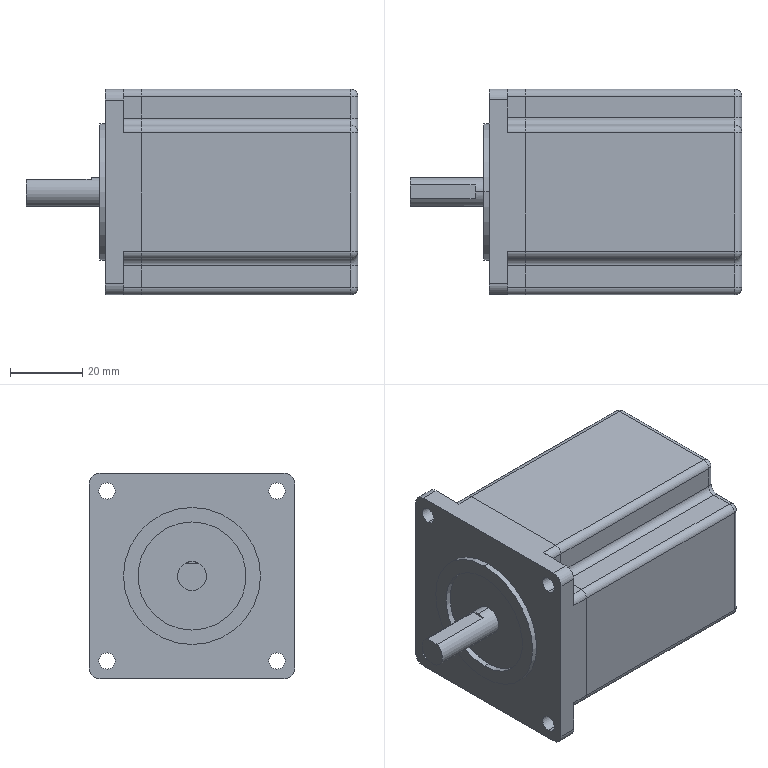Component | SolidWorks | 57Stepper-1 | 2 solids | 103 faces | box 92 x 57 x 57 mm | volume 202432 mm3 | cylinder 54 | plane 37 | sphere 8 | torus 4 | commonest cylinder face diameters 4 x36 4.5 x8 6 x4 8 x2 30 x2 38 x2
build123d program:
from build123d import *

# Parameters (mm, degrees)
SKETCH1_W           = 57
SKETCH1_H           = 57
BOSS_EXTRUDE1_DEPTH = 10
SKETCH2_R           = 19
SKETCH2_R_2         = 15
BOSS_EXTRUDE2_DEPTH = 1.6
FILLET1_R           = 3
SKETCH3_R           = 4
BOSS_EXTRUDE3_DEPTH = 22
SKETCH4_W           = 15
SKETCH4_H           = 15
CUT_EXTRUDE1_DEPTH  = 5
FILLET2_R           = 2
BOSS_EXTRUDE4_DEPTH = 60
FILLET3_R           = 2
SKETCH7_R           = 2.25
CUT_EXTRUDE2_DEPTH  = 77.482
CIRPATTERN1_COUNT   = 4
SKETCH8_W           = 3
SKETCH8_H           = 10
CUT_EXTRUDE3_DEPTH  = 18


with BuildPart() as part:
    # Sketch1 → Boss-Extrude1 (new body)
    with BuildSketch(Plane(origin=(0, 0, 0), x_dir=(0, 0, -1), z_dir=(1, 0, 0))):
        Rectangle(SKETCH1_W, SKETCH1_H)
    extrude(amount=BOSS_EXTRUDE1_DEPTH)

    # Sketch2 → Boss-Extrude2 (add)
    with BuildSketch(Plane(origin=(10, 0, 0), x_dir=(0, 0, -1), z_dir=(1, 0, 0))):
        Circle(SKETCH2_R)
        Circle(SKETCH2_R_2, mode=Mode.SUBTRACT)
    extrude(amount=BOSS_EXTRUDE2_DEPTH)

    # Fillet1
    fillet1_edges = [part.edges().sort_by_distance(p)[0] for p in [
        (5, -28.5, -28.5),
        (5, -28.5, 28.5),
        (5, 28.5, 28.5),
        (5, 28.5, -28.5),
    ]]
    fillet(fillet1_edges, radius=FILLET1_R)

    # Sketch3 → Boss-Extrude3 (add)
    with BuildSketch(Plane(origin=(10, 0, 0), x_dir=(0, 0, -1), z_dir=(1, 0, 0))):
        Circle(SKETCH3_R)
    extrude(amount=BOSS_EXTRUDE3_DEPTH)

    # Sketch4 → Cut-Extrude1 (cut)
    with BuildSketch(Plane.ZY):
        with Locations((26, 26)):
            Rectangle(SKETCH4_W, SKETCH4_H)
        with Locations((26, -26)):
            Rectangle(SKETCH4_W, SKETCH4_H)
        with Locations((-26, -26)):
            Rectangle(SKETCH4_W, SKETCH4_H)
        with Locations((-26, 26)):
            Rectangle(SKETCH4_W, SKETCH4_H)
    extrude(amount=-CUT_EXTRUDE1_DEPTH, mode=Mode.SUBTRACT)

    # Fillet2
    fillet2_edges = [part.edges().sort_by_distance(p)[0] for p in [
        (2.5, 18.5, -28.5),
        (2.5, 18.5, -18.5),
        (2.5, 28.5, -18.5),
        (2.5, 28.5, 18.5),
        (2.5, 18.5, 18.5),
        (2.5, 18.5, 28.5),
        (2.5, -18.5, 28.5),
        (2.5, -18.5, 18.5),
        (2.5, -28.5, 18.5),
        (2.5, -28.5, -18.5),
        (2.5, -18.5, -18.5),
        (2.5, -18.5, -28.5),
    ]]
    fillet(fillet2_edges, radius=FILLET2_R)

    # Sketch7 → Cut-Extrude2 (cut, through all)
    with BuildSketch(Plane.ZY.offset(-5)):
        with Locations((-23.57, 23.57)):
            Circle(SKETCH7_R)
    cut_extrude2 = extrude(amount=-CUT_EXTRUDE2_DEPTH, mode=Mode.SUBTRACT)

    # CirPattern1: Cut-Extrude2 ×4 about axis
    cirpattern1_axis = Axis((0, 0, 0), (1, 0, 0))
    for i in range(1, CIRPATTERN1_COUNT):
        add(cut_extrude2.rotate(cirpattern1_axis, i * 360 / CIRPATTERN1_COUNT), mode=Mode.SUBTRACT)

    # Sketch8 → Cut-Extrude3 (cut)
    with BuildSketch(Plane(origin=(32, 0, 0), x_dir=(0, 0, -1), z_dir=(1, 0, 0))):
        with Locations((5, 0)):
            Rectangle(SKETCH8_W, SKETCH8_H)
    extrude(amount=-CUT_EXTRUDE3_DEPTH, mode=Mode.SUBTRACT)


with BuildPart() as body_2:
    # Sketch6 → Boss-Extrude4 (new body)
    with BuildSketch(Plane.ZY):
        with BuildLine():
            Line((-18.5, 26.5), (-18.5, 20.5))
            ThreePointArc((-18.5, 20.5), (-19.086, 19.086), (-20.5, 18.5))
            Line((-20.5, 18.5), (-26.5, 18.5))
            ThreePointArc((-26.5, 18.5), (-27.914, 17.914), (-28.5, 16.5))
            Line((-28.5, 16.5), (-28.5, -16.5))
            ThreePointArc((-28.5, -16.5), (-27.914, -17.914), (-26.5, -18.5))
            Line((-26.5, -18.5), (-20.5, -18.5))
            ThreePointArc((-20.5, -18.5), (-19.086, -19.086), (-18.5, -20.5))
            Line((-18.5, -20.5), (-18.5, -26.5))
            ThreePointArc((-18.5, -26.5), (-17.914, -27.914), (-16.5, -28.5))
            Line((-16.5, -28.5), (16.5, -28.5))
            ThreePointArc((16.5, -28.5), (17.914, -27.914), (18.5, -26.5))
            Line((18.5, -26.5), (18.5, -20.5))
            ThreePointArc((18.5, -20.5), (19.086, -19.086), (20.5, -18.5))
            Line((20.5, -18.5), (26.5, -18.5))
            ThreePointArc((26.5, -18.5), (27.914, -17.914), (28.5, -16.5))
            Line((28.5, -16.5), (28.5, 16.5))
            ThreePointArc((28.5, 16.5), (27.914, 17.914), (26.5, 18.5))
            Line((26.5, 18.5), (20.5, 18.5))
            ThreePointArc((20.5, 18.5), (19.086, 19.086), (18.5, 20.5))
            Line((18.5, 20.5), (18.5, 26.5))
            ThreePointArc((18.5, 26.5), (17.914, 27.914), (16.5, 28.5))
            Line((16.5, 28.5), (-16.5, 28.5))
            ThreePointArc((-16.5, 28.5), (-17.914, 27.914), (-18.5, 26.5))
        make_face()
    extrude(amount=BOSS_EXTRUDE4_DEPTH)

    # Fillet3
    fillet3_edges = [body_2.edges().sort_by_distance(p)[0] for p in [
        (-60, 19.086, 19.086),
        (-60, 23.5, 18.5),
        (-60, 27.914, 17.914),
        (-60, 28.5, 0),
        (-60, 27.914, -17.914),
        (-60, 23.5, -18.5),
        (-60, 19.086, -19.086),
        (-60, 18.5, -23.5),
        (-60, 17.914, -27.914),
        (-60, 0, -28.5),
        (-60, 17.914, 27.914),
        (-60, -17.914, -27.914),
        (-60, -18.5, -23.5),
        (-60, -19.086, -19.086),
        (-60, -23.5, -18.5),
        (-60, -27.914, -17.914),
        (-60, -28.5, 0),
        (-60, -27.914, 17.914),
        (-60, -23.5, 18.5),
        (-60, -19.086, 19.086),
        (-60, -18.5, 23.5),
        (-60, 18.5, 23.5),
        (-60, -17.914, 27.914),
        (-60, 0, 28.5),
    ]]
    fillet(fillet3_edges, radius=FILLET3_R)


solid = Compound([part.part, body_2.part])

# Placed as in the assembly
solid = solid.moved(Location((4, -99.859, 124.987), (-180, 0, 180)))